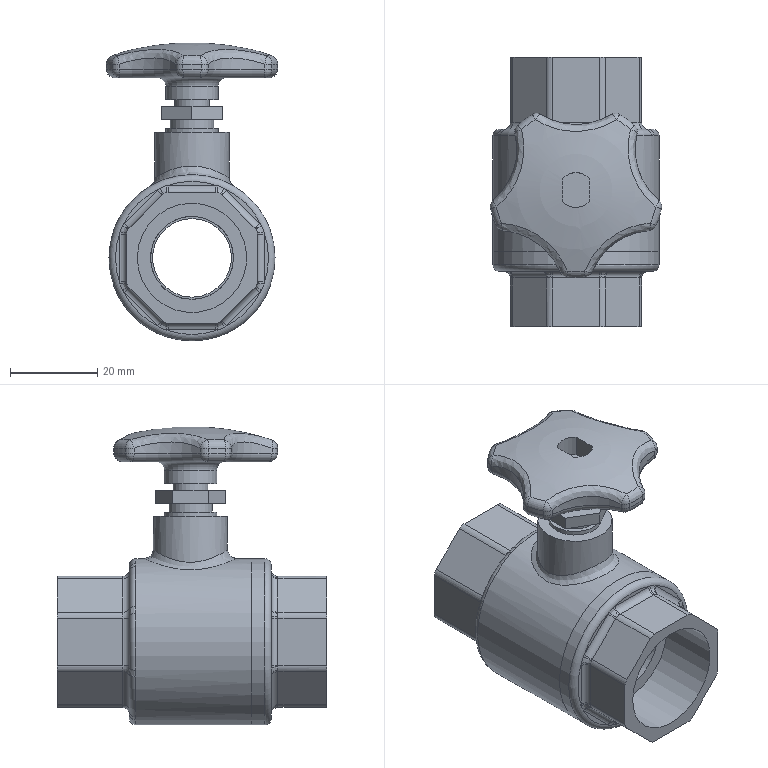Assembly | NX | mm | 9 component files | 9 solids | 259 faces | box 39.21 x 61.7 x 68.12 mm | volume 41144 mm3 | cylinder 82 | plane 80 | torus 49 | sphere 24 | spline 22 | cone 2 | commonest cylinder face diameters 4 x26 3 x16 8 x6 40 x5 30 x5 12 x4 26 x4 10 x3
Bill of materials:
unnamed part 1 | 1 |  | Hollow, rotationally based fitting-like body: an octagonal prism section with a round through-bore, a wider round flange collar with a filleted transition, and a short plain cylindrical spigot on the far side.
unnamed part 2 | 1 |  | Stepped cylindrical shaft/pin: a long main cylinder with a flat cut near its upper end (D-shaped top end), a slightly smaller upper step, a larger collar near the lower end, and a short lower section that has a flat face and a smaller stub.
unnamed part 3 | 1 |  | Tee-shaped hollow body: a large thin-walled cylindrical sleeve with a round through-bore, a smaller hollow cylindrical branch boss standing perpendicular on its side with a filleted joint, and a stepped-down polygonal (hex-like) section at one end of the main axis.
unnamed part 4 | 2 |  | Thin flat annular ring (washer-like) with a rectangular cross-section and a small chamfer on the outer edge.
unnamed part 5 | 1 |  | Bushing-like part with a hexagonal flange at one end, a round through-bore, a narrow reduced-diameter neck/undercut below the hex, and a larger plain cylindrical body.
unnamed part 6 | 1 |  | Plain thick-walled cylindrical ring/sleeve with a concentric round through-bore and flat end faces.
unnamed part 7 | 1 |  | Spherical body with a large cylindrical through-bore, two parallel flat truncations at the bore ends, and a rectangular slot cut across the top perpendicular to the bore.
unnamed part 8 | 1 |  | Five-lobed star-shaped grip knob with a domed top, rounded edges, concave scallops between the lobes, a cylindrical hub underneath, and a central double-D (obround with flats) through-hole.
Mates:
1. concentric | valve_bonnet 1 edge | valve_body 1 edge
2. concentric | seal_ring 2 edge | valve_bonnet 1 edge
3. concentric | seal_ring 1 edge | valve_body 1 edge
4. touch align | valve_core 1 face | valve_bonnet 1 face
5. center | valve_stem 1 face | valve_stem 1 face | valve_core 1 face | valve_core 1 face
6. concentric | valve_stem 1 edge | valve_body 1 edge
7. concentric | packing 1 edge | valve_body 1 edge
8. concentric | packing_gland 1 edge | packing 1 edge
9. concentric | knob 1 edge | valve_stem 1 edge